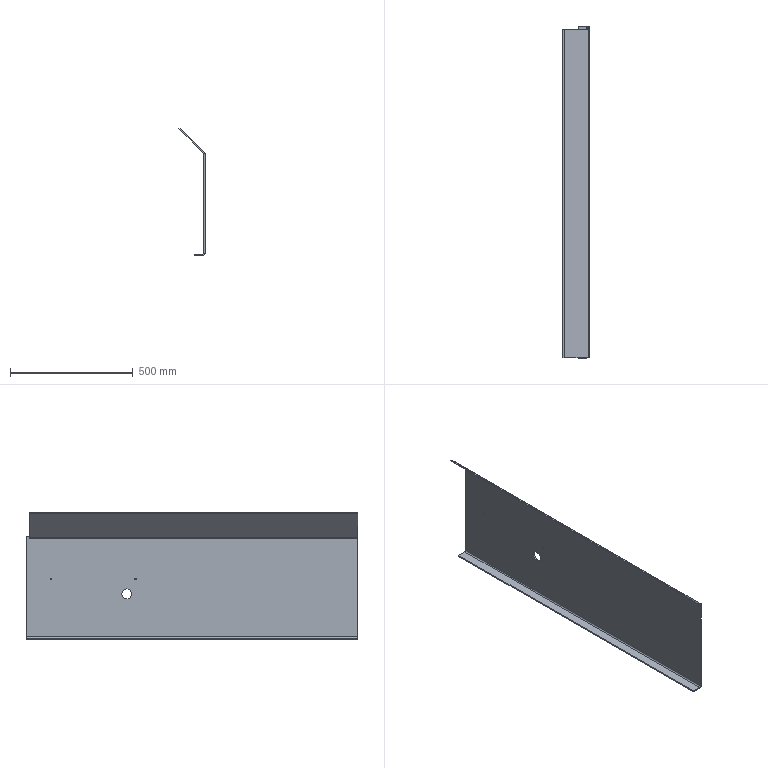Component | SolidWorks | 005FrameSheet-MetalB-1 | 2 solids | 26 faces | box 107.07 x 1350 x 515 mm | volume 3987894 mm3 | plane 16 | cylinder 10 | commonest cylinder face diameters 5 x4 40 x2 10 x2 20 x2 | material Plain Carbon Steel
build123d program:
from build123d import *

# Parameters (mm, degrees)
SKETCH2_W                  = 410
SKETCH2_H                  = 515
BOSS_EXTRUDE1_DEPTH        = 1350
FILLET1_R                  = 10
CHAMFER1_SIZE              = 100
FILLET2_R                  = 10
SHELL1_T                   = -5
CUT_EXTRUDE1_REACH         = 1461.366
SKETCH3_W                  = 320
SKETCH3_H                  = 1561.085
SKETCH7_R                  = 13
SKETCH7_R_2                = 3.25
CUT_EXTRUDE5_DEPTH         = 5
SKETCH8_R                  = 7.5
CUT_EXTRUDE6_DEPTH         = 5
M6_TAPPED_HOLE1_AT_2_COUNT = 2
M6_TAPPED_HOLE1_AT_2_PITCH = 60
LPATTERN1_COUNT            = 2
LPATTERN1_PITCH            = 345
SKETCH13_R                 = 20
CUT_EXTRUDE7_DEPTH         = 5
M6_TAPPED_HOLE3_AT_2_COUNT = 2
M6_TAPPED_HOLE3_AT_2_PITCH = 60
CUT_EXTRUDE9_DEPTH         = 1390.544
SKETCH18_W                 = 400
SKETCH18_H                 = 30
CUT_EXTRUDE10_DEPTH        = 1390.544
CUT_EXTRUDE8_DEPTH         = 1390.544
CUT_EXTRUDE8_DEPTH_BACK    = 1390.544
SKETCH16_W                 = 227.729
SKETCH16_H                 = 1450
BOSS_EXTRUDE2_DEPTH        = 1335


with BuildPart() as part:
    # Sketch2 → Boss-Extrude1 (new body)
    with BuildSketch(Plane(origin=(0, 0, 0), x_dir=(1, 0, 0), z_dir=(0, 1, 0))):
        Rectangle(SKETCH2_W, SKETCH2_H)
    extrude(amount=BOSS_EXTRUDE1_DEPTH)

    # Fillet1
    fillet1_edges = [part.edges().sort_by_distance(p)[0] for p in [
        (-205, 675, -257.5),
        (205, 675, -257.5),
    ]]
    fillet(fillet1_edges, radius=FILLET1_R)

    # Chamfer1
    chamfer1_edges = [part.edges().sort_by_distance(p)[0] for p in [
        (205, 675, 257.5),
        (-205, 675, 257.5),
    ]]
    chamfer(chamfer1_edges, length=CHAMFER1_SIZE)

    # Fillet2
    fillet2_edges = [part.edges().sort_by_distance(p)[0] for p in [
        (205, 675, 157.5),
        (-205, 675, 157.5),
    ]]
    fillet(fillet2_edges, radius=FILLET2_R)

    # Shell1
    shell1_openings = [part.faces().sort_by_distance(p)[0] for p in [
        (0, 1350, -11.096),
        (0, 0, -11.096),
        (0, 675, 257.5),
    ]]
    offset(amount=SHELL1_T, openings=shell1_openings, kind=Kind.INTERSECTION)

    # Sketch3 → Cut-Extrude1 (cut, up to next)
    with BuildSketch(Plane(origin=(0, 0, -257.5), x_dir=(-1, 0, 0), z_dir=(0, 0, -1)), mode=Mode.PRIVATE) as cut_extrude1_sk1:
        with Locations((0, 708.71)):
            Rectangle(SKETCH3_W, SKETCH3_H)
    cut_extrude1_tool1 = extrude(cut_extrude1_sk1.sketch, amount=-CUT_EXTRUDE1_REACH, mode=Mode.PRIVATE) & part.part
    add(cut_extrude1_tool1.solids().sort_by_distance((0, 708.71, -257.5))[0], mode=Mode.SUBTRACT)


with BuildPart() as cut_extrude1_piece_1:
    # of the separate pieces the step leaves, piece 1, a body of its own (cut_extrude1_pieces)
    add(part.part.solids().sort_by_distance((195, 0, -257.5))[0])

    # Sketch11 → M6 Tapped Hole2 (revolve, cut)
    with BuildSketch(Plane(origin=(205, 1250, -12.5), x_dir=(0, 0, -1), z_dir=(0, 1, 0))):
        Polygon((0, 0), (0, 16.502), (2.5, 15), (2.5, 0), align=None)
    m6_tapped_hole2 = revolve(axis=Axis((211.35, 1250, -12.5), (-1, 0, 0)), mode=Mode.SUBTRACT)

    # LPattern1: M6 Tapped Hole2 ×2
    with Locations(*[(0, -i * LPATTERN1_PITCH, 0) for i in range(1, LPATTERN1_COUNT)]):
        add(m6_tapped_hole2, mode=Mode.SUBTRACT)

    # Sketch13 → Cut-Extrude7 (cut)
    with BuildSketch(Plane(origin=(205, 0, 0), x_dir=(0, 0, -1), z_dir=(1, 0, 0))):
        with Locations((72.5, 940)):
            Circle(SKETCH13_R)
    extrude(amount=-CUT_EXTRUDE7_DEPTH, mode=Mode.SUBTRACT)


with BuildPart() as cut_extrude1_piece_2:
    # of the separate pieces the step leaves, piece 2, a body of its own (cut_extrude1_pieces)
    add(part.part.solids().sort_by_distance((-202.071, 0, 160.429))[0])

    # Sketch7 → Cut-Extrude5 (cut)
    with BuildSketch(Plane.ZY.offset(205)):
        with Locations((-151.5, 191.5)):
            Circle(SKETCH7_R)
        with Locations((-151.5, 318.5)):
            Circle(SKETCH7_R)
        with Locations((-151.5, 293)):
            Circle(SKETCH7_R_2)
        with Locations((-151.5, 217)):
            Circle(SKETCH7_R_2)
        with Locations((-93.5, 191.5)):
            Circle(SKETCH7_R)
        with Locations((-93.5, 318.5)):
            Circle(SKETCH7_R)
        with Locations((-93.5, 217)):
            Circle(SKETCH7_R_2)
        with Locations((-93.5, 293)):
            Circle(SKETCH7_R_2)
    extrude(amount=-CUT_EXTRUDE5_DEPTH, mode=Mode.SUBTRACT)

    # Sketch8 → Cut-Extrude6 (cut)
    with BuildSketch(Plane.ZY.offset(205)):
        with Locations((-147.5, 95)):
            Circle(SKETCH8_R)
        with Locations((-97.5, 95)):
            Circle(SKETCH8_R)
        with Locations((-147.5, 65)):
            Circle(SKETCH8_R)
        with Locations((-97.5, 65)):
            Circle(SKETCH8_R)
    extrude(amount=-CUT_EXTRUDE6_DEPTH, mode=Mode.SUBTRACT)

    # Sketch9 → M6 Tapped Hole1 (revolve, cut)
    with BuildSketch(Plane(origin=(-205, 80, -92.5), x_dir=(0, 0, 1), z_dir=(0, 1, 0))):
        Polygon((0, 0), (0, 16.502), (2.5, 15), (2.5, 0), align=None)
    m6_tapped_hole1 = revolve(axis=Axis((-211.35, 80, -92.5), (1, 0, 0)), mode=Mode.SUBTRACT)

    # M6 Tapped Hole1 at 2: M6 Tapped Hole1 ×2
    with Locations(*[(0, 0, -i * M6_TAPPED_HOLE1_AT_2_PITCH) for i in range(1, M6_TAPPED_HOLE1_AT_2_COUNT)]):
        add(m6_tapped_hole1, mode=Mode.SUBTRACT)

    # Sketch14 → M6 Tapped Hole3 (revolve, cut)
    with BuildSketch(Plane(origin=(-205, 1250, 100), x_dir=(0, 0, 1), z_dir=(0, 1, 0))):
        Polygon((0, 0), (0, 16.502), (2.5, 15), (2.5, 0), align=None)
    m6_tapped_hole3 = revolve(axis=Axis((-211.35, 1250, 100), (1, 0, 0)), mode=Mode.SUBTRACT)

    # M6 Tapped Hole3 at 2: M6 Tapped Hole3 ×2
    with Locations(*[(0, 0, i * M6_TAPPED_HOLE3_AT_2_PITCH) for i in range(1, M6_TAPPED_HOLE3_AT_2_COUNT)]):
        add(m6_tapped_hole3, mode=Mode.SUBTRACT)


with BuildPart() as cut_extrude9_tool:
    # Sketch17 → Cut-Extrude9 (new, through all)
    with BuildSketch(Plane(origin=(0, 1350, 0), x_dir=(1, 0, 0), z_dir=(0, 1, 0))):
        Polygon((-105, -257.5), (0, -152.5), (105, -257.5), align=None)
    extrude(amount=-CUT_EXTRUDE9_DEPTH)


with BuildPart() as cut_extrude1_piece_1_1:
    add(cut_extrude1_piece_1.part)

    # Cut-Extrude9: cut by cut_extrude9_tool
    add(cut_extrude9_tool.part, mode=Mode.SUBTRACT)


with BuildPart() as cut_extrude1_piece_2_1:
    add(cut_extrude1_piece_2.part)

    # Cut-Extrude9: cut by cut_extrude9_tool
    add(cut_extrude9_tool.part, mode=Mode.SUBTRACT)


with BuildPart() as cut_extrude10_tool:
    # Sketch18 → Cut-Extrude10 (new, through all)
    with BuildSketch(Plane.XY):
        with Locations((0, 1350)):
            Rectangle(SKETCH18_W, SKETCH18_H)
    extrude(amount=CUT_EXTRUDE10_DEPTH)


with BuildPart() as cut_extrude1_piece_1_2:
    add(cut_extrude1_piece_1_1.part)

    # Cut-Extrude10: cut by cut_extrude10_tool
    add(cut_extrude10_tool.part, mode=Mode.SUBTRACT)


with BuildPart() as cut_extrude1_piece_2_2:
    add(cut_extrude1_piece_2_1.part)

    # Cut-Extrude10: cut by cut_extrude10_tool
    add(cut_extrude10_tool.part, mode=Mode.SUBTRACT)

    # Sketch16 → Cut-Extrude8 (cut, two sides: drawn at the far end of the back side and taken through both)
    with BuildSketch(Plane.XY.offset(-CUT_EXTRUDE8_DEPTH_BACK)):
        with Locations((-113.864, 725)):
            Rectangle(SKETCH16_W, SKETCH16_H)
    extrude(amount=CUT_EXTRUDE8_DEPTH + CUT_EXTRUDE8_DEPTH_BACK, mode=Mode.SUBTRACT)


with BuildPart() as body_2:
    # Sketch19 → Boss-Extrude2 (new, through all)
    with BuildSketch(Plane(origin=(0, 1335, 0), x_dir=(1, 0, 0), z_dir=(0, 1, 0))):
        Polygon((105, -257.5), (101.464, -253.964), (97.929, -257.5), align=None)
    extrude(amount=-BOSS_EXTRUDE2_DEPTH)


solid = Compound([cut_extrude1_piece_1_2.part, body_2.part])

# Placed as in the assembly
solid = solid.moved(Location((100, 37, -262.5), (0, 0, 0)))
STEP:
#1=COLOUR_RGB('',0.7922,0.8196,0.9333);
#2=FILL_AREA_STYLE_COLOUR('',#1);
#3=FILL_AREA_STYLE('',(#2));
#4=SURFACE_STYLE_FILL_AREA(#3);
#5=SURFACE_SIDE_STYLE('',(#4));
#6=SURFACE_STYLE_USAGE(.BOTH.,#5);
#7=PRESENTATION_STYLE_ASSIGNMENT((#6));
#8=CARTESIAN_POINT('',(11.811,38.465,-12.402));
#9=VERTEX_POINT('',#8);
#10=CARTESIAN_POINT('',(11.811,38.465,-13.976));
#11=VERTEX_POINT('',#10);
#12=CARTESIAN_POINT('',(11.811,38.465,-13.189));
#13=DIRECTION('',(1.,0.,0.));
#14=DIRECTION('',(0.,0.,1.));
#15=AXIS2_PLACEMENT_3D('',#12,#13,#14);
#16=CIRCLE('',#15,0.7874);
#17=EDGE_CURVE('',#9,#11,#16,.T.);
#18=ORIENTED_EDGE('',*,*,#17,.F.);
#19=CARTESIAN_POINT('',(12.008,38.465,-12.402));
#20=VERTEX_POINT('',#19);
#21=CARTESIAN_POINT('',(-4.134,38.465,-12.402));
#22=DIRECTION('',(1.,0.,0.));
#23=VECTOR('',#22,39.37);
#24=LINE('',#21,#23);
#25=EDGE_CURVE('',#9,#20,#24,.T.);
#26=ORIENTED_EDGE('',*,*,#25,.T.);
#27=CARTESIAN_POINT('',(12.008,38.465,-13.976));
#28=VERTEX_POINT('',#27);
#29=CARTESIAN_POINT('',(12.008,38.465,-13.189));
#30=DIRECTION('',(1.,0.,0.));
#31=DIRECTION('',(0.,0.,-1.));
#32=AXIS2_PLACEMENT_3D('',#29,#30,#31);
#33=CIRCLE('',#32,0.7874);
#34=EDGE_CURVE('',#20,#28,#33,.T.);
#35=ORIENTED_EDGE('',*,*,#34,.T.);
#36=CARTESIAN_POINT('',(-4.134,38.465,-13.976));
#37=DIRECTION('',(1.,0.,0.));
#38=VECTOR('',#37,39.37);
#39=LINE('',#36,#38);
#40=EDGE_CURVE('',#11,#28,#39,.T.);
#41=ORIENTED_EDGE('',*,*,#40,.F.);
#42=EDGE_LOOP('',(#18,#26,#35,#41));
#43=FACE_OUTER_BOUND('',#42,.T.);
#44=CARTESIAN_POINT('',(-4.134,38.465,-13.189));
#45=DIRECTION('',(1.,0.,0.));
#46=DIRECTION('',(0.,0.,-1.));
#47=AXIS2_PLACEMENT_3D('',#44,#45,#46);
#48=CYLINDRICAL_SURFACE('',#47,0.7874);
#49=ADVANCED_FACE('',(#43),#48,.F.);
#50=CARTESIAN_POINT('',(11.811,37.087,-10.925));
#51=VERTEX_POINT('',#50);
#52=CARTESIAN_POINT('',(11.811,37.087,-10.728));
#53=VERTEX_POINT('',#52);
#54=CARTESIAN_POINT('',(11.811,37.087,-10.827));
#55=DIRECTION('',(-1.,0.,0.));
#56=DIRECTION('',(0.,0.,1.));
#57=AXIS2_PLACEMENT_3D('',#54,#55,#56);
#58=CIRCLE('',#57,0.09843);
#59=EDGE_CURVE('',#51,#53,#58,.T.);
#60=ORIENTED_EDGE('',*,*,#59,.T.);
#61=CARTESIAN_POINT('',(12.008,37.087,-10.728));
#62=VERTEX_POINT('',#61);
#63=CARTESIAN_POINT('',(12.008,37.087,-10.728));
#64=DIRECTION('',(1.,0.,0.));
#65=VECTOR('',#64,39.37);
#66=LINE('',#63,#65);
#67=EDGE_CURVE('',#53,#62,#66,.T.);
#68=ORIENTED_EDGE('',*,*,#67,.T.);
#69=CARTESIAN_POINT('',(12.008,37.087,-10.925));
#70=VERTEX_POINT('',#69);
#71=CARTESIAN_POINT('',(12.008,37.087,-10.827));
#72=DIRECTION('',(1.,0.,0.));
#73=DIRECTION('',(0.,0.,-1.));
#74=AXIS2_PLACEMENT_3D('',#71,#72,#73);
#75=CIRCLE('',#74,0.09843);
#76=EDGE_CURVE('',#62,#70,#75,.T.);
#77=ORIENTED_EDGE('',*,*,#76,.T.);
#78=CARTESIAN_POINT('',(12.008,37.087,-10.925));
#79=DIRECTION('',(1.,0.,0.));
#80=VECTOR('',#79,39.37);
#81=LINE('',#78,#80);
#82=EDGE_CURVE('',#51,#70,#81,.T.);
#83=ORIENTED_EDGE('',*,*,#82,.F.);
#84=EDGE_LOOP('',(#60,#68,#77,#83));
#85=FACE_OUTER_BOUND('',#84,.T.);
#86=CARTESIAN_POINT('',(12.008,37.087,-10.827));
#87=DIRECTION('',(1.,0.,0.));
#88=DIRECTION('',(0.,0.,-1.));
#89=AXIS2_PLACEMENT_3D('',#86,#87,#88);
#90=CYLINDRICAL_SURFACE('',#89,0.09843);
#91=ADVANCED_FACE('',(#85),#90,.F.);
#92=CARTESIAN_POINT('',(11.811,50.669,-10.925));
#93=VERTEX_POINT('',#92);
#94=CARTESIAN_POINT('',(11.811,50.669,-10.728));
#95=VERTEX_POINT('',#94);
#96=CARTESIAN_POINT('',(11.811,50.669,-10.827));
#97=DIRECTION('',(-1.,0.,0.));
#98=DIRECTION('',(0.,0.,1.));
#99=AXIS2_PLACEMENT_3D('',#96,#97,#98);
#100=CIRCLE('',#99,0.09843);
#101=EDGE_CURVE('',#93,#95,#100,.T.);
#102=ORIENTED_EDGE('',*,*,#101,.T.);
#103=CARTESIAN_POINT('',(12.008,50.669,-10.728));
#104=VERTEX_POINT('',#103);
#105=CARTESIAN_POINT('',(12.008,50.669,-10.728));
#106=DIRECTION('',(1.,0.,0.));
#107=VECTOR('',#106,39.37);
#108=LINE('',#105,#107);
#109=EDGE_CURVE('',#95,#104,#108,.T.);
#110=ORIENTED_EDGE('',*,*,#109,.T.);
#111=CARTESIAN_POINT('',(12.008,50.669,-10.925));
#112=VERTEX_POINT('',#111);
#113=CARTESIAN_POINT('',(12.008,50.669,-10.827));
#114=DIRECTION('',(1.,0.,0.));
#115=DIRECTION('',(0.,0.,-1.));
#116=AXIS2_PLACEMENT_3D('',#113,#114,#115);
#117=CIRCLE('',#116,0.09843);
#118=EDGE_CURVE('',#104,#112,#117,.T.);
#119=ORIENTED_EDGE('',*,*,#118,.T.);
#120=CARTESIAN_POINT('',(12.008,50.669,-10.925));
#121=DIRECTION('',(1.,0.,0.));
#122=VECTOR('',#121,39.37);
#123=LINE('',#120,#122);
#124=EDGE_CURVE('',#93,#112,#123,.T.);
#125=ORIENTED_EDGE('',*,*,#124,.F.);
#126=EDGE_LOOP('',(#102,#110,#119,#125));
#127=FACE_OUTER_BOUND('',#126,.T.);
#128=CARTESIAN_POINT('',(12.008,50.669,-10.827));
#129=DIRECTION('',(1.,0.,0.));
#130=DIRECTION('',(0.,0.,-1.));
#131=AXIS2_PLACEMENT_3D('',#128,#129,#130);
#132=CYLINDRICAL_SURFACE('',#131,0.09843);
#133=ADVANCED_FACE('',(#127),#132,.F.);
#134=CARTESIAN_POINT('',(11.811,54.606,-3.937));
#135=VERTEX_POINT('',#134);
#136=CARTESIAN_POINT('',(11.811,54.606,-20.079));
#137=VERTEX_POINT('',#136);
#138=CARTESIAN_POINT('',(11.811,54.606,-20.472));
#139=DIRECTION('',(0.,0.,-1.));
#140=VECTOR('',#139,39.37);
#141=LINE('',#138,#140);
#142=EDGE_CURVE('',#135,#137,#141,.T.);
#143=ORIENTED_EDGE('',*,*,#142,.F.);
#144=CARTESIAN_POINT('',(11.893,54.606,-4.019));
#145=VERTEX_POINT('',#144);
#146=CARTESIAN_POINT('',(12.008,54.606,-4.134));
#147=DIRECTION('',(0.7071,0.,-0.7071));
#148=VECTOR('',#147,39.37);
#149=LINE('',#146,#148);
#150=EDGE_CURVE('',#135,#145,#149,.T.);
#151=ORIENTED_EDGE('',*,*,#150,.T.);
#152=CARTESIAN_POINT('',(12.008,54.606,-4.297));
#153=VERTEX_POINT('',#152);
#154=CARTESIAN_POINT('',(11.614,54.606,-4.297));
#155=DIRECTION('',(0.,1.,0.));
#156=DIRECTION('',(-0.,0.,-1.));
#157=AXIS2_PLACEMENT_3D('',#154,#155,#156);
#158=CIRCLE('',#157,0.3937);
#159=EDGE_CURVE('',#145,#153,#158,.T.);
#160=ORIENTED_EDGE('',*,*,#159,.T.);
#161=CARTESIAN_POINT('',(12.008,54.606,-20.079));
#162=VERTEX_POINT('',#161);
#163=CARTESIAN_POINT('',(12.008,54.606,-0.1969));
#164=DIRECTION('',(0.,0.,-1.));
#165=VECTOR('',#164,39.37);
#166=LINE('',#163,#165);
#167=EDGE_CURVE('',#153,#162,#166,.T.);
#168=ORIENTED_EDGE('',*,*,#167,.T.);
#169=CARTESIAN_POINT('',(11.614,54.606,-20.472));
#170=VERTEX_POINT('',#169);
#171=CARTESIAN_POINT('',(11.614,54.606,-20.079));
#172=DIRECTION('',(0.,1.,0.));
#173=DIRECTION('',(0.,0.,-1.));
#174=AXIS2_PLACEMENT_3D('',#171,#172,#173);
#175=CIRCLE('',#174,0.3937);
#176=EDGE_CURVE('',#162,#170,#175,.T.);
#177=ORIENTED_EDGE('',*,*,#176,.T.);
#178=CARTESIAN_POINT('',(10.236,54.606,-20.472));
#179=VERTEX_POINT('',#178);
#180=CARTESIAN_POINT('',(-4.134,54.606,-20.472));
#181=DIRECTION('',(-1.,0.,0.));
#182=VECTOR('',#181,39.37);
#183=LINE('',#180,#182);
#184=EDGE_CURVE('',#170,#179,#183,.T.);
#185=ORIENTED_EDGE('',*,*,#184,.T.);
#186=CARTESIAN_POINT('',(10.236,54.606,-20.276));
#187=VERTEX_POINT('',#186);
#188=CARTESIAN_POINT('',(10.236,54.606,-0.1968));
#189=DIRECTION('',(0.,0.,-1.));
#190=VECTOR('',#189,39.37);
#191=LINE('',#188,#190);
#192=EDGE_CURVE('',#187,#179,#191,.T.);
#193=ORIENTED_EDGE('',*,*,#192,.F.);
#194=CARTESIAN_POINT('',(11.614,54.606,-20.276));
#195=VERTEX_POINT('',#194);
#196=CARTESIAN_POINT('',(12.008,54.606,-20.276));
#197=DIRECTION('',(-1.,0.,0.));
#198=VECTOR('',#197,39.37);
#199=LINE('',#196,#198);
#200=EDGE_CURVE('',#195,#187,#199,.T.);
#201=ORIENTED_EDGE('',*,*,#200,.F.);
#202=CARTESIAN_POINT('',(11.614,54.606,-20.079));
#203=DIRECTION('',(0.,1.,0.));
#204=DIRECTION('',(0.,0.,-1.));
#205=AXIS2_PLACEMENT_3D('',#202,#203,#204);
#206=CIRCLE('',#205,0.1969);
#207=EDGE_CURVE('',#137,#195,#206,.T.);
#208=ORIENTED_EDGE('',*,*,#207,.F.);
#209=EDGE_LOOP('',(#143,#151,#160,#168,#177,#185,#193,#201,#208));
#210=FACE_OUTER_BOUND('',#209,.T.);
#211=CARTESIAN_POINT('',(12.008,54.606,-20.472));
#212=DIRECTION('',(0.,-1.,0.));
#213=DIRECTION('',(0.,0.,-1.));
#214=AXIS2_PLACEMENT_3D('',#211,#212,#213);
#215=PLANE('',#214);
#216=ADVANCED_FACE('',(#210),#215,.F.);
#217=CARTESIAN_POINT('',(11.811,54.016,-3.937));
#218=VERTEX_POINT('',#217);
#219=CARTESIAN_POINT('',(11.811,54.606,-3.937));
#220=DIRECTION('',(0.,-1.,0.));
#221=VECTOR('',#220,39.37);
#222=LINE('',#219,#221);
#223=EDGE_CURVE('',#135,#218,#222,.T.);
#224=ORIENTED_EDGE('',*,*,#223,.T.);
#225=CARTESIAN_POINT('',(8.071,54.016,-0.1969));
#226=VERTEX_POINT('',#225);
#227=CARTESIAN_POINT('',(12.008,54.016,-4.134));
#228=DIRECTION('',(-0.7071,0.,0.7071));
#229=VECTOR('',#228,39.37);
#230=LINE('',#227,#229);
#231=EDGE_CURVE('',#218,#226,#230,.T.);
#232=ORIENTED_EDGE('',*,*,#231,.T.);
#233=CARTESIAN_POINT('',(8.071,1.457,-0.1969));
#234=VERTEX_POINT('',#233);
#235=CARTESIAN_POINT('',(8.071,54.606,-0.1969));
#236=DIRECTION('',(0.,1.,0.));
#237=VECTOR('',#236,39.37);
#238=LINE('',#235,#237);
#239=EDGE_CURVE('',#234,#226,#238,.T.);
#240=ORIENTED_EDGE('',*,*,#239,.F.);
#241=CARTESIAN_POINT('',(11.893,1.457,-4.019));
#242=VERTEX_POINT('',#241);
#243=CARTESIAN_POINT('',(20.177,1.457,-12.303));
#244=DIRECTION('',(-0.7071,0.,0.7071));
#245=VECTOR('',#244,39.37);
#246=LINE('',#243,#245);
#247=EDGE_CURVE('',#242,#234,#246,.T.);
#248=ORIENTED_EDGE('',*,*,#247,.F.);
#249=CARTESIAN_POINT('',(11.893,54.606,-4.019));
#250=DIRECTION('',(0.,1.,0.));
#251=VECTOR('',#250,39.37);
#252=LINE('',#249,#251);
#253=EDGE_CURVE('',#242,#145,#252,.T.);
#254=ORIENTED_EDGE('',*,*,#253,.T.);
#255=ORIENTED_EDGE('',*,*,#150,.F.);
#256=EDGE_LOOP('',(#224,#232,#240,#248,#254,#255));
#257=FACE_OUTER_BOUND('',#256,.T.);
#258=CARTESIAN_POINT('',(12.008,54.606,-4.134));
#259=DIRECTION('',(-0.7071,0.,-0.7071));
#260=DIRECTION('',(-0.7071,0.,0.7071));
#261=AXIS2_PLACEMENT_3D('',#258,#259,#260);
#262=PLANE('',#261);
#263=ADVANCED_FACE('',(#257),#262,.F.);
#264=CARTESIAN_POINT('',(11.753,54.016,-4.158));
#265=VERTEX_POINT('',#264);
#266=CARTESIAN_POINT('',(7.932,54.016,-0.336));
#267=VERTEX_POINT('',#266);
#268=CARTESIAN_POINT('',(11.869,54.016,-4.273));
#269=DIRECTION('',(-0.7071,0.,0.7071));
#270=VECTOR('',#269,39.37);
#271=LINE('',#268,#270);
#272=EDGE_CURVE('',#265,#267,#271,.T.);
#273=ORIENTED_EDGE('',*,*,#272,.F.);
#274=CARTESIAN_POINT('',(11.753,1.457,-4.158));
#275=VERTEX_POINT('',#274);
#276=CARTESIAN_POINT('',(11.753,54.606,-4.158));
#277=DIRECTION('',(0.,1.,0.));
#278=VECTOR('',#277,39.37);
#279=LINE('',#276,#278);
#280=EDGE_CURVE('',#275,#265,#279,.T.);
#281=ORIENTED_EDGE('',*,*,#280,.F.);
#282=CARTESIAN_POINT('',(7.932,1.457,-0.336));
#283=VERTEX_POINT('',#282);
#284=CARTESIAN_POINT('',(20.038,1.457,-12.442));
#285=DIRECTION('',(-0.7071,0.,0.7071));
#286=VECTOR('',#285,39.37);
#287=LINE('',#284,#286);
#288=EDGE_CURVE('',#275,#283,#287,.T.);
#289=ORIENTED_EDGE('',*,*,#288,.T.);
#290=CARTESIAN_POINT('',(7.932,54.606,-0.336));
#291=DIRECTION('',(0.,1.,0.));
#292=VECTOR('',#291,39.37);
#293=LINE('',#290,#292);
#294=EDGE_CURVE('',#283,#267,#293,.T.);
#295=ORIENTED_EDGE('',*,*,#294,.T.);
#296=EDGE_LOOP('',(#273,#281,#289,#295));
#297=FACE_OUTER_BOUND('',#296,.T.);
#298=CARTESIAN_POINT('',(11.869,54.606,-4.273));
#299=DIRECTION('',(-0.7071,0.,-0.7071));
#300=DIRECTION('',(-0.7071,0.,0.7071));
#301=AXIS2_PLACEMENT_3D('',#298,#299,#300);
#302=PLANE('',#301);
#303=ADVANCED_FACE('',(#297),#302,.T.);
#304=CARTESIAN_POINT('',(11.811,54.016,-4.297));
#305=VERTEX_POINT('',#304);
#306=CARTESIAN_POINT('',(11.614,54.016,-4.297));
#307=DIRECTION('',(0.,-1.,0.));
#308=DIRECTION('',(0.,0.,1.));
#309=AXIS2_PLACEMENT_3D('',#306,#307,#308);
#310=CIRCLE('',#309,0.1969);
#311=EDGE_CURVE('',#305,#265,#310,.T.);
#312=ORIENTED_EDGE('',*,*,#311,.F.);
#313=CARTESIAN_POINT('',(11.811,1.457,-4.297));
#314=VERTEX_POINT('',#313);
#315=CARTESIAN_POINT('',(11.811,54.606,-4.297));
#316=DIRECTION('',(0.,-1.,0.));
#317=VECTOR('',#316,39.37);
#318=LINE('',#315,#317);
#319=EDGE_CURVE('',#305,#314,#318,.T.);
#320=ORIENTED_EDGE('',*,*,#319,.T.);
#321=CARTESIAN_POINT('',(11.614,1.457,-4.297));
#322=DIRECTION('',(0.,-1.,0.));
#323=DIRECTION('',(0.,0.,-1.));
#324=AXIS2_PLACEMENT_3D('',#321,#322,#323);
#325=CIRCLE('',#324,0.1969);
#326=EDGE_CURVE('',#314,#275,#325,.T.);
#327=ORIENTED_EDGE('',*,*,#326,.T.);
#328=ORIENTED_EDGE('',*,*,#280,.T.);
#329=EDGE_LOOP('',(#312,#320,#327,#328));
#330=FACE_OUTER_BOUND('',#329,.T.);
#331=CARTESIAN_POINT('',(11.614,54.606,-4.297));
#332=DIRECTION('',(0.,-1.,0.));
#333=DIRECTION('',(0.,0.,-1.));
#334=AXIS2_PLACEMENT_3D('',#331,#332,#333);
#335=CYLINDRICAL_SURFACE('',#334,0.1969);
#336=ADVANCED_FACE('',(#330),#335,.F.);
#337=CARTESIAN_POINT('',(3.937,54.016,-4.331));
#338=DIRECTION('',(0.7071,0.,0.7071));
#339=VECTOR('',#338,39.37);
#340=LINE('',#337,#339);
#341=EDGE_CURVE('',#267,#226,#340,.T.);
#342=ORIENTED_EDGE('',*,*,#341,.F.);
#343=ORIENTED_EDGE('',*,*,#294,.F.);
#344=CARTESIAN_POINT('',(3.937,1.457,-4.331));
#345=DIRECTION('',(-0.7071,0.,-0.7071));
#346=VECTOR('',#345,39.37);
#347=LINE('',#344,#346);
#348=EDGE_CURVE('',#234,#283,#347,.T.);
#349=ORIENTED_EDGE('',*,*,#348,.F.);
#350=ORIENTED_EDGE('',*,*,#239,.T.);
#351=EDGE_LOOP('',(#342,#343,#349,#350));
#352=FACE_OUTER_BOUND('',#351,.T.);
#353=CARTESIAN_POINT('',(3.937,1.457,-4.331));
#354=DIRECTION('',(0.7071,0.,-0.7071));
#355=DIRECTION('',(-0.7071,0.,-0.7071));
#356=AXIS2_PLACEMENT_3D('',#353,#354,#355);
#357=PLANE('',#356);
#358=ADVANCED_FACE('',(#352),#357,.F.);
#359=CARTESIAN_POINT('',(11.614,1.457,-20.472));
#360=VERTEX_POINT('',#359);
#361=CARTESIAN_POINT('',(10.236,1.457,-20.472));
#362=VERTEX_POINT('',#361);
#363=CARTESIAN_POINT('',(-4.134,1.457,-20.472));
#364=DIRECTION('',(-1.,0.,0.));
#365=VECTOR('',#364,39.37);
#366=LINE('',#363,#365);
#367=EDGE_CURVE('',#360,#362,#366,.T.);
#368=ORIENTED_EDGE('',*,*,#367,.T.);
#369=CARTESIAN_POINT('',(10.236,60.089,-20.472));
#370=DIRECTION('',(-0.,-1.,0.));
#371=VECTOR('',#370,39.37);
#372=LINE('',#369,#371);
#373=EDGE_CURVE('',#179,#362,#372,.T.);
#374=ORIENTED_EDGE('',*,*,#373,.F.);
#375=ORIENTED_EDGE('',*,*,#184,.F.);
#376=CARTESIAN_POINT('',(11.614,54.606,-20.472));
#377=DIRECTION('',(0.,-1.,0.));
#378=VECTOR('',#377,39.37);
#379=LINE('',#376,#378);
#380=EDGE_CURVE('',#170,#360,#379,.T.);
#381=ORIENTED_EDGE('',*,*,#380,.T.);
#382=EDGE_LOOP('',(#368,#374,#375,#381));
#383=FACE_OUTER_BOUND('',#382,.T.);
#384=CARTESIAN_POINT('',(-4.134,54.606,-20.472));
#385=DIRECTION('',(0.,0.,1.));
#386=DIRECTION('',(1.,0.,0.));
#387=AXIS2_PLACEMENT_3D('',#384,#385,#386);
#388=PLANE('',#387);
#389=ADVANCED_FACE('',(#383),#388,.F.);
#390=ORIENTED_EDGE('',*,*,#348,.T.);
#391=ORIENTED_EDGE('',*,*,#288,.F.);
#392=ORIENTED_EDGE('',*,*,#326,.F.);
#393=CARTESIAN_POINT('',(11.811,1.457,-20.079));
#394=VERTEX_POINT('',#393);
#395=CARTESIAN_POINT('',(11.811,1.457,-20.472));
#396=DIRECTION('',(0.,0.,-1.));
#397=VECTOR('',#396,39.37);
#398=LINE('',#395,#397);
#399=EDGE_CURVE('',#314,#394,#398,.T.);
#400=ORIENTED_EDGE('',*,*,#399,.T.);
#401=CARTESIAN_POINT('',(11.614,1.457,-20.276));
#402=VERTEX_POINT('',#401);
#403=CARTESIAN_POINT('',(11.614,1.457,-20.079));
#404=DIRECTION('',(0.,-1.,0.));
#405=DIRECTION('',(0.,0.,-1.));
#406=AXIS2_PLACEMENT_3D('',#403,#404,#405);
#407=CIRCLE('',#406,0.1969);
#408=EDGE_CURVE('',#402,#394,#407,.T.);
#409=ORIENTED_EDGE('',*,*,#408,.F.);
#410=CARTESIAN_POINT('',(10.236,1.457,-20.276));
#411=VERTEX_POINT('',#410);
#412=CARTESIAN_POINT('',(12.008,1.457,-20.276));
#413=DIRECTION('',(-1.,0.,0.));
#414=VECTOR('',#413,39.37);
#415=LINE('',#412,#414);
#416=EDGE_CURVE('',#402,#411,#415,.T.);
#417=ORIENTED_EDGE('',*,*,#416,.T.);
#418=CARTESIAN_POINT('',(10.236,1.457,-0.1968));
#419=DIRECTION('',(0.,0.,-1.));
#420=VECTOR('',#419,39.37);
#421=LINE('',#418,#420);
#422=EDGE_CURVE('',#411,#362,#421,.T.);
#423=ORIENTED_EDGE('',*,*,#422,.T.);
#424=ORIENTED_EDGE('',*,*,#367,.F.);
#425=CARTESIAN_POINT('',(12.008,1.457,-20.079));
#426=VERTEX_POINT('',#425);
#427=CARTESIAN_POINT('',(11.614,1.457,-20.079));
#428=DIRECTION('',(0.,-1.,0.));
#429=DIRECTION('',(0.,0.,-1.));
#430=AXIS2_PLACEMENT_3D('',#427,#428,#429);
#431=CIRCLE('',#430,0.3937);
#432=EDGE_CURVE('',#360,#426,#431,.T.);
#433=ORIENTED_EDGE('',*,*,#432,.T.);
#434=CARTESIAN_POINT('',(12.008,1.457,-4.297));
#435=VERTEX_POINT('',#434);
#436=CARTESIAN_POINT('',(12.008,1.457,-0.1969));
#437=DIRECTION('',(0.,0.,-1.));
#438=VECTOR('',#437,39.37);
#439=LINE('',#436,#438);
#440=EDGE_CURVE('',#435,#426,#439,.T.);
#441=ORIENTED_EDGE('',*,*,#440,.F.);
#442=CARTESIAN_POINT('',(11.614,1.457,-4.297));
#443=DIRECTION('',(0.,-1.,0.));
#444=DIRECTION('',(0.,0.,-1.));
#445=AXIS2_PLACEMENT_3D('',#442,#443,#444);
#446=CIRCLE('',#445,0.3937);
#447=EDGE_CURVE('',#435,#242,#446,.T.);
#448=ORIENTED_EDGE('',*,*,#447,.T.);
#449=ORIENTED_EDGE('',*,*,#247,.T.);
#450=EDGE_LOOP('',(#390,#391,#392,#400,#409,#417,#423,#424,#433,#441,#448,#449));
#451=FACE_OUTER_BOUND('',#450,.T.);
#452=CARTESIAN_POINT('',(12.008,1.457,-20.472));
#453=DIRECTION('',(0.,-1.,0.));
#454=DIRECTION('',(0.,0.,-1.));
#455=AXIS2_PLACEMENT_3D('',#452,#453,#454);
#456=PLANE('',#455);
#457=ADVANCED_FACE('',(#451),#456,.T.);
#458=CARTESIAN_POINT('',(10.236,60.089,-20.276));
#459=DIRECTION('',(-0.,-1.,0.));
#460=VECTOR('',#459,39.37);
#461=LINE('',#458,#460);
#462=EDGE_CURVE('',#187,#411,#461,.T.);
#463=ORIENTED_EDGE('',*,*,#462,.T.);
#464=ORIENTED_EDGE('',*,*,#416,.F.);
#465=CARTESIAN_POINT('',(11.614,54.606,-20.276));
#466=DIRECTION('',(0.,-1.,0.));
#467=VECTOR('',#466,39.37);
#468=LINE('',#465,#467);
#469=EDGE_CURVE('',#195,#402,#468,.T.);
#470=ORIENTED_EDGE('',*,*,#469,.F.);
#471=ORIENTED_EDGE('',*,*,#200,.T.);
#472=EDGE_LOOP('',(#463,#464,#470,#471));
#473=FACE_OUTER_BOUND('',#472,.T.);
#474=CARTESIAN_POINT('',(-4.134,54.606,-20.276));
#475=DIRECTION('',(0.,0.,1.));
#476=DIRECTION('',(1.,0.,0.));
#477=AXIS2_PLACEMENT_3D('',#474,#475,#476);
#478=PLANE('',#477);
#479=ADVANCED_FACE('',(#473),#478,.T.);
#480=CARTESIAN_POINT('',(12.008,38.465,-13.189));
#481=DIRECTION('',(1.,0.,0.));
#482=DIRECTION('',(0.,0.,-1.));
#483=AXIS2_PLACEMENT_3D('',#480,#481,#482);
#484=CIRCLE('',#483,0.7874);
#485=EDGE_CURVE('',#28,#20,#484,.T.);
#486=ORIENTED_EDGE('',*,*,#485,.F.);
#487=ORIENTED_EDGE('',*,*,#34,.F.);
#488=EDGE_LOOP('',(#486,#487));
#489=FACE_BOUND('',#488,.T.);
#490=CARTESIAN_POINT('',(12.008,37.087,-10.827));
#491=DIRECTION('',(1.,0.,0.));
#492=DIRECTION('',(0.,0.,-1.));
#493=AXIS2_PLACEMENT_3D('',#490,#491,#492);
#494=CIRCLE('',#493,0.09843);
#495=EDGE_CURVE('',#70,#62,#494,.T.);
#496=ORIENTED_EDGE('',*,*,#495,.F.);
#497=ORIENTED_EDGE('',*,*,#76,.F.);
#498=EDGE_LOOP('',(#496,#497));
#499=FACE_BOUND('',#498,.T.);
#500=CARTESIAN_POINT('',(12.008,50.669,-10.827));
#501=DIRECTION('',(1.,0.,0.));
#502=DIRECTION('',(0.,0.,-1.));
#503=AXIS2_PLACEMENT_3D('',#500,#501,#502);
#504=CIRCLE('',#503,0.09843);
#505=EDGE_CURVE('',#112,#104,#504,.T.);
#506=ORIENTED_EDGE('',*,*,#505,.F.);
#507=ORIENTED_EDGE('',*,*,#118,.F.);
#508=EDGE_LOOP('',(#506,#507));
#509=FACE_BOUND('',#508,.T.);
#510=ORIENTED_EDGE('',*,*,#167,.F.);
#511=CARTESIAN_POINT('',(12.008,1.457,-4.297));
#512=DIRECTION('',(0.,-1.,0.));
#513=VECTOR('',#512,39.37);
#514=LINE('',#511,#513);
#515=EDGE_CURVE('',#153,#435,#514,.T.);
#516=ORIENTED_EDGE('',*,*,#515,.T.);
#517=ORIENTED_EDGE('',*,*,#440,.T.);
#518=CARTESIAN_POINT('',(12.008,54.606,-20.079));
#519=DIRECTION('',(0.,1.,0.));
#520=VECTOR('',#519,39.37);
#521=LINE('',#518,#520);
#522=EDGE_CURVE('',#426,#162,#521,.T.);
#523=ORIENTED_EDGE('',*,*,#522,.T.);
#524=EDGE_LOOP('',(#510,#516,#517,#523));
#525=FACE_OUTER_BOUND('',#524,.T.);
#526=CARTESIAN_POINT('',(12.008,54.606,-0.1969));
#527=DIRECTION('',(-1.,0.,0.));
#528=DIRECTION('',(0.,0.,1.));
#529=AXIS2_PLACEMENT_3D('',#526,#527,#528);
#530=PLANE('',#529);
#531=ADVANCED_FACE('',(#489,#499,#509,#525),#530,.F.);
#532=ORIENTED_EDGE('',*,*,#176,.F.);
#533=ORIENTED_EDGE('',*,*,#522,.F.);
#534=ORIENTED_EDGE('',*,*,#432,.F.);
#535=ORIENTED_EDGE('',*,*,#380,.F.);
#536=EDGE_LOOP('',(#532,#533,#534,#535));
#537=FACE_OUTER_BOUND('',#536,.T.);
#538=CARTESIAN_POINT('',(11.614,54.606,-20.079));
#539=DIRECTION('',(0.,-1.,0.));
#540=DIRECTION('',(0.,0.,-1.));
#541=AXIS2_PLACEMENT_3D('',#538,#539,#540);
#542=CYLINDRICAL_SURFACE('',#541,0.3937);
#543=ADVANCED_FACE('',(#537),#542,.T.);
#544=ORIENTED_EDGE('',*,*,#159,.F.);
#545=ORIENTED_EDGE('',*,*,#253,.F.);
#546=ORIENTED_EDGE('',*,*,#447,.F.);
#547=ORIENTED_EDGE('',*,*,#515,.F.);
#548=EDGE_LOOP('',(#544,#545,#546,#547));
#549=FACE_OUTER_BOUND('',#548,.T.);
#550=CARTESIAN_POINT('',(11.614,54.606,-4.297));
#551=DIRECTION('',(0.,-1.,0.));
#552=DIRECTION('',(0.,0.,-1.));
#553=AXIS2_PLACEMENT_3D('',#550,#551,#552);
#554=CYLINDRICAL_SURFACE('',#553,0.3937);
#555=ADVANCED_FACE('',(#549),#554,.T.);
#556=ORIENTED_EDGE('',*,*,#319,.F.);
#557=CARTESIAN_POINT('',(11.811,54.016,-0.1969));
#558=DIRECTION('',(0.,0.,-1.));
#559=VECTOR('',#558,39.37);
#560=LINE('',#557,#559);
#561=EDGE_CURVE('',#218,#305,#560,.T.);
#562=ORIENTED_EDGE('',*,*,#561,.F.);
#563=ORIENTED_EDGE('',*,*,#223,.F.);
#564=ORIENTED_EDGE('',*,*,#142,.T.);
#565=CARTESIAN_POINT('',(11.811,54.606,-20.079));
#566=DIRECTION('',(0.,1.,0.));
#567=VECTOR('',#566,39.37);
#568=LINE('',#565,#567);
#569=EDGE_CURVE('',#394,#137,#568,.T.);
#570=ORIENTED_EDGE('',*,*,#569,.F.);
#571=ORIENTED_EDGE('',*,*,#399,.F.);
#572=EDGE_LOOP('',(#556,#562,#563,#564,#570,#571));
#573=FACE_OUTER_BOUND('',#572,.T.);
#574=CARTESIAN_POINT('',(11.811,38.465,-13.189));
#575=DIRECTION('',(1.,0.,0.));
#576=DIRECTION('',(0.,0.,1.));
#577=AXIS2_PLACEMENT_3D('',#574,#575,#576);
#578=CIRCLE('',#577,0.7874);
#579=EDGE_CURVE('',#11,#9,#578,.T.);
#580=ORIENTED_EDGE('',*,*,#579,.T.);
#581=ORIENTED_EDGE('',*,*,#17,.T.);
#582=EDGE_LOOP('',(#580,#581));
#583=FACE_BOUND('',#582,.T.);
#584=ORIENTED_EDGE('',*,*,#59,.F.);
#585=CARTESIAN_POINT('',(11.811,37.087,-10.827));
#586=DIRECTION('',(-1.,0.,0.));
#587=DIRECTION('',(0.,0.,1.));
#588=AXIS2_PLACEMENT_3D('',#585,#586,#587);
#589=CIRCLE('',#588,0.09843);
#590=EDGE_CURVE('',#53,#51,#589,.T.);
#591=ORIENTED_EDGE('',*,*,#590,.F.);
#592=EDGE_LOOP('',(#584,#591));
#593=FACE_BOUND('',#592,.T.);
#594=ORIENTED_EDGE('',*,*,#101,.F.);
#595=CARTESIAN_POINT('',(11.811,50.669,-10.827));
#596=DIRECTION('',(-1.,0.,0.));
#597=DIRECTION('',(0.,0.,1.));
#598=AXIS2_PLACEMENT_3D('',#595,#596,#597);
#599=CIRCLE('',#598,0.09843);
#600=EDGE_CURVE('',#95,#93,#599,.T.);
#601=ORIENTED_EDGE('',*,*,#600,.F.);
#602=EDGE_LOOP('',(#594,#601));
#603=FACE_BOUND('',#602,.T.);
#604=CARTESIAN_POINT('',(11.811,54.606,-0.1969));
#605=DIRECTION('',(-1.,0.,0.));
#606=DIRECTION('',(0.,0.,1.));
#607=AXIS2_PLACEMENT_3D('',#604,#605,#606);
#608=PLANE('',#607);
#609=ADVANCED_FACE('',(#573,#583,#593,#603),#608,.T.);
#610=ORIENTED_EDGE('',*,*,#207,.T.);
#611=ORIENTED_EDGE('',*,*,#469,.T.);
#612=ORIENTED_EDGE('',*,*,#408,.T.);
#613=ORIENTED_EDGE('',*,*,#569,.T.);
#614=EDGE_LOOP('',(#610,#611,#612,#613));
#615=FACE_OUTER_BOUND('',#614,.T.);
#616=CARTESIAN_POINT('',(11.614,54.606,-20.079));
#617=DIRECTION('',(0.,-1.,0.));
#618=DIRECTION('',(0.,0.,-1.));
#619=AXIS2_PLACEMENT_3D('',#616,#617,#618);
#620=CYLINDRICAL_SURFACE('',#619,0.1969);
#621=ADVANCED_FACE('',(#615),#620,.F.);
#622=ORIENTED_EDGE('',*,*,#192,.T.);
#623=ORIENTED_EDGE('',*,*,#373,.T.);
#624=ORIENTED_EDGE('',*,*,#422,.F.);
#625=ORIENTED_EDGE('',*,*,#462,.F.);
#626=EDGE_LOOP('',(#622,#623,#624,#625));
#627=FACE_OUTER_BOUND('',#626,.T.);
#628=CARTESIAN_POINT('',(10.236,60.089,-0.1968));
#629=DIRECTION('',(1.,-0.,0.));
#630=DIRECTION('',(0.,1.,0.));
#631=AXIS2_PLACEMENT_3D('',#628,#629,#630);
#632=PLANE('',#631);
#633=ADVANCED_FACE('',(#627),#632,.F.);
#634=ORIENTED_EDGE('',*,*,#109,.F.);
#635=ORIENTED_EDGE('',*,*,#600,.T.);
#636=ORIENTED_EDGE('',*,*,#124,.T.);
#637=ORIENTED_EDGE('',*,*,#505,.T.);
#638=EDGE_LOOP('',(#634,#635,#636,#637));
#639=FACE_OUTER_BOUND('',#638,.T.);
#640=CARTESIAN_POINT('',(12.008,50.669,-10.827));
#641=DIRECTION('',(1.,0.,0.));
#642=DIRECTION('',(0.,0.,-1.));
#643=AXIS2_PLACEMENT_3D('',#640,#641,#642);
#644=CYLINDRICAL_SURFACE('',#643,0.09843);
#645=ADVANCED_FACE('',(#639),#644,.F.);
#646=ORIENTED_EDGE('',*,*,#67,.F.);
#647=ORIENTED_EDGE('',*,*,#590,.T.);
#648=ORIENTED_EDGE('',*,*,#82,.T.);
#649=ORIENTED_EDGE('',*,*,#495,.T.);
#650=EDGE_LOOP('',(#646,#647,#648,#649));
#651=FACE_OUTER_BOUND('',#650,.T.);
#652=CARTESIAN_POINT('',(12.008,37.087,-10.827));
#653=DIRECTION('',(1.,0.,0.));
#654=DIRECTION('',(0.,0.,-1.));
#655=AXIS2_PLACEMENT_3D('',#652,#653,#654);
#656=CYLINDRICAL_SURFACE('',#655,0.09843);
#657=ADVANCED_FACE('',(#651),#656,.F.);
#658=ORIENTED_EDGE('',*,*,#25,.F.);
#659=ORIENTED_EDGE('',*,*,#579,.F.);
#660=ORIENTED_EDGE('',*,*,#40,.T.);
#661=ORIENTED_EDGE('',*,*,#485,.T.);
#662=EDGE_LOOP('',(#658,#659,#660,#661));
#663=FACE_OUTER_BOUND('',#662,.T.);
#664=CARTESIAN_POINT('',(-4.134,38.465,-13.189));
#665=DIRECTION('',(1.,0.,0.));
#666=DIRECTION('',(0.,0.,-1.));
#667=AXIS2_PLACEMENT_3D('',#664,#665,#666);
#668=CYLINDRICAL_SURFACE('',#667,0.7874);
#669=ADVANCED_FACE('',(#663),#668,.F.);
#670=ORIENTED_EDGE('',*,*,#311,.T.);
#671=ORIENTED_EDGE('',*,*,#272,.T.);
#672=ORIENTED_EDGE('',*,*,#341,.T.);
#673=ORIENTED_EDGE('',*,*,#231,.F.);
#674=ORIENTED_EDGE('',*,*,#561,.T.);
#675=EDGE_LOOP('',(#670,#671,#672,#673,#674));
#676=FACE_OUTER_BOUND('',#675,.T.);
#677=CARTESIAN_POINT('',(-3.937,54.016,-0.1969));
#678=DIRECTION('',(0.,1.,0.));
#679=DIRECTION('',(0.,0.,1.));
#680=AXIS2_PLACEMENT_3D('',#677,#678,#679);
#681=PLANE('',#680);
#682=ADVANCED_FACE('',(#676),#681,.T.);
#683=CLOSED_SHELL('',(#49,#91,#133,#216,#263,#303,#336,#358,#389,#457,#479,#531,#543,#555,#609,#621,#633,#645,#657,#669,#682));
#684=MANIFOLD_SOLID_BREP('',#683);
#685=STYLED_ITEM('',(#7),#684);
#686=PRESENTATION_LAYER_ASSIGNMENT('','',(#685));
#687=COLOUR_RGB('',0.7922,0.8196,0.9333);
#688=FILL_AREA_STYLE_COLOUR('',#687);
#689=FILL_AREA_STYLE('',(#688));
#690=SURFACE_STYLE_FILL_AREA(#689);
#691=SURFACE_SIDE_STYLE('',(#690));
#692=SURFACE_STYLE_USAGE(.BOTH.,#691);
#693=PRESENTATION_STYLE_ASSIGNMENT((#692));
#694=CARTESIAN_POINT('',(7.792,54.016,-0.1969));
#695=VERTEX_POINT('',#694);
#696=CARTESIAN_POINT('',(8.071,54.016,-0.1969));
#697=VERTEX_POINT('',#696);
#698=CARTESIAN_POINT('',(7.792,54.016,-0.1969));
#699=DIRECTION('',(1.,0.,0.));
#700=VECTOR('',#699,39.37);
#701=LINE('',#698,#700);
#702=EDGE_CURVE('',#695,#697,#701,.T.);
#703=ORIENTED_EDGE('',*,*,#702,.F.);
#704=CARTESIAN_POINT('',(7.792,1.457,-0.1969));
#705=VERTEX_POINT('',#704);
#706=CARTESIAN_POINT('',(7.792,1.457,-0.1969));
#707=DIRECTION('',(0.,1.,0.));
#708=VECTOR('',#707,39.37);
#709=LINE('',#706,#708);
#710=EDGE_CURVE('',#705,#695,#709,.T.);
#711=ORIENTED_EDGE('',*,*,#710,.F.);
#712=CARTESIAN_POINT('',(8.071,1.457,-0.1969));
#713=VERTEX_POINT('',#712);
#714=CARTESIAN_POINT('',(7.792,1.457,-0.1969));
#715=DIRECTION('',(1.,0.,0.));
#716=VECTOR('',#715,39.37);
#717=LINE('',#714,#716);
#718=EDGE_CURVE('',#705,#713,#717,.T.);
#719=ORIENTED_EDGE('',*,*,#718,.T.);
#720=CARTESIAN_POINT('',(8.071,1.457,-0.1969));
#721=DIRECTION('',(0.,1.,0.));
#722=VECTOR('',#721,39.37);
#723=LINE('',#720,#722);
#724=EDGE_CURVE('',#713,#697,#723,.T.);
#725=ORIENTED_EDGE('',*,*,#724,.T.);
#726=EDGE_LOOP('',(#703,#711,#719,#725));
#727=FACE_OUTER_BOUND('',#726,.T.);
#728=CARTESIAN_POINT('',(7.792,1.457,-0.1969));
#729=DIRECTION('',(0.,0.,1.));
#730=DIRECTION('',(1.,0.,0.));
#731=AXIS2_PLACEMENT_3D('',#728,#729,#730);
#732=PLANE('',#731);
#733=ADVANCED_FACE('',(#727),#732,.T.);
#734=CARTESIAN_POINT('',(7.932,54.016,-0.336));
#735=VERTEX_POINT('',#734);
#736=CARTESIAN_POINT('',(7.932,54.016,-0.336));
#737=DIRECTION('',(-0.7071,0.,0.7071));
#738=VECTOR('',#737,39.37);
#739=LINE('',#736,#738);
#740=EDGE_CURVE('',#735,#695,#739,.T.);
#741=ORIENTED_EDGE('',*,*,#740,.F.);
#742=CARTESIAN_POINT('',(7.932,1.457,-0.336));
#743=VERTEX_POINT('',#742);
#744=CARTESIAN_POINT('',(7.932,1.457,-0.336));
#745=DIRECTION('',(0.,1.,0.));
#746=VECTOR('',#745,39.37);
#747=LINE('',#744,#746);
#748=EDGE_CURVE('',#743,#735,#747,.T.);
#749=ORIENTED_EDGE('',*,*,#748,.F.);
#750=CARTESIAN_POINT('',(7.932,1.457,-0.336));
#751=DIRECTION('',(-0.7071,0.,0.7071));
#752=VECTOR('',#751,39.37);
#753=LINE('',#750,#752);
#754=EDGE_CURVE('',#743,#705,#753,.T.);
#755=ORIENTED_EDGE('',*,*,#754,.T.);
#756=ORIENTED_EDGE('',*,*,#710,.T.);
#757=EDGE_LOOP('',(#741,#749,#755,#756));
#758=FACE_OUTER_BOUND('',#757,.T.);
#759=CARTESIAN_POINT('',(7.932,1.457,-0.336));
#760=DIRECTION('',(-0.7071,0.,-0.7071));
#761=DIRECTION('',(-0.7071,0.,0.7071));
#762=AXIS2_PLACEMENT_3D('',#759,#760,#761);
#763=PLANE('',#762);
#764=ADVANCED_FACE('',(#758),#763,.T.);
#765=CARTESIAN_POINT('',(8.071,54.016,-0.1969));
#766=DIRECTION('',(-0.7071,0.,-0.7071));
#767=VECTOR('',#766,39.37);
#768=LINE('',#765,#767);
#769=EDGE_CURVE('',#697,#735,#768,.T.);
#770=ORIENTED_EDGE('',*,*,#769,.F.);
#771=ORIENTED_EDGE('',*,*,#724,.F.);
#772=CARTESIAN_POINT('',(8.071,1.457,-0.1969));
#773=DIRECTION('',(-0.7071,0.,-0.7071));
#774=VECTOR('',#773,39.37);
#775=LINE('',#772,#774);
#776=EDGE_CURVE('',#713,#743,#775,.T.);
#777=ORIENTED_EDGE('',*,*,#776,.T.);
#778=ORIENTED_EDGE('',*,*,#748,.T.);
#779=EDGE_LOOP('',(#770,#771,#777,#778));
#780=FACE_OUTER_BOUND('',#779,.T.);
#781=CARTESIAN_POINT('',(8.071,1.457,-0.1969));
#782=DIRECTION('',(0.7071,0.,-0.7071));
#783=DIRECTION('',(-0.7071,0.,-0.7071));
#784=AXIS2_PLACEMENT_3D('',#781,#782,#783);
#785=PLANE('',#784);
#786=ADVANCED_FACE('',(#780),#785,.T.);
#787=ORIENTED_EDGE('',*,*,#718,.F.);
#788=ORIENTED_EDGE('',*,*,#754,.F.);
#789=ORIENTED_EDGE('',*,*,#776,.F.);
#790=EDGE_LOOP('',(#787,#788,#789));
#791=FACE_OUTER_BOUND('',#790,.T.);
#792=CARTESIAN_POINT('',(8.071,1.457,-0.1969));
#793=DIRECTION('',(0.,1.,0.));
#794=DIRECTION('',(0.,0.,1.));
#795=AXIS2_PLACEMENT_3D('',#792,#793,#794);
#796=PLANE('',#795);
#797=ADVANCED_FACE('',(#791),#796,.F.);
#798=ORIENTED_EDGE('',*,*,#702,.T.);
#799=ORIENTED_EDGE('',*,*,#769,.T.);
#800=ORIENTED_EDGE('',*,*,#740,.T.);
#801=EDGE_LOOP('',(#798,#799,#800));
#802=FACE_OUTER_BOUND('',#801,.T.);
#803=CARTESIAN_POINT('',(8.071,54.016,-0.1969));
#804=DIRECTION('',(0.,1.,0.));
#805=DIRECTION('',(0.,0.,1.));
#806=AXIS2_PLACEMENT_3D('',#803,#804,#805);
#807=PLANE('',#806);
#808=ADVANCED_FACE('',(#802),#807,.T.);
#809=CLOSED_SHELL('',(#733,#764,#786,#797,#808));
#810=MANIFOLD_SOLID_BREP('',#809);
#811=STYLED_ITEM('',(#693),#810);
#812=(LENGTH_UNIT()NAMED_UNIT(*)SI_UNIT($,.METRE.));
#813=LENGTH_MEASURE_WITH_UNIT(LENGTH_MEASURE(0.0254),#812);
#814=DIMENSIONAL_EXPONENTS(1.,0.,0.,0.,0.,0.,0.);
#815=(CONVERSION_BASED_UNIT('',#813)LENGTH_UNIT()NAMED_UNIT(#814));
#816=UNCERTAINTY_MEASURE_WITH_UNIT(LENGTH_MEASURE(0.00001),#815,'','');
#817=(NAMED_UNIT(*)PLANE_ANGLE_UNIT()SI_UNIT($,.RADIAN.));
#818=(NAMED_UNIT(*)SI_UNIT($,.STERADIAN.)SOLID_ANGLE_UNIT());
#819=(GEOMETRIC_REPRESENTATION_CONTEXT(3)GLOBAL_UNCERTAINTY_ASSIGNED_CONTEXT((#816))GLOBAL_UNIT_ASSIGNED_CONTEXT((#815,#817,#818))REPRESENTATION_CONTEXT('',''));
#820=MECHANICAL_DESIGN_GEOMETRIC_PRESENTATION_REPRESENTATION('',(#811),#819);
#821=CARTESIAN_POINT('',(0.,0.,0.));
#822=DIRECTION('',(0.,0.,1.));
#823=DIRECTION('',(1.,0.,0.));
#824=AXIS2_PLACEMENT_3D('',#821,#822,#823);
#825=(LENGTH_UNIT()NAMED_UNIT(*)SI_UNIT($,.METRE.));
#826=LENGTH_MEASURE_WITH_UNIT(LENGTH_MEASURE(0.0254),#825);
#827=DIMENSIONAL_EXPONENTS(1.,0.,0.,0.,0.,0.,0.);
#828=(CONVERSION_BASED_UNIT('',#826)LENGTH_UNIT()NAMED_UNIT(#827));
#829=UNCERTAINTY_MEASURE_WITH_UNIT(LENGTH_MEASURE(0.00001),#828,'','');
#830=(NAMED_UNIT(*)PLANE_ANGLE_UNIT()SI_UNIT($,.RADIAN.));
#831=(NAMED_UNIT(*)SI_UNIT($,.STERADIAN.)SOLID_ANGLE_UNIT());
#832=(GEOMETRIC_REPRESENTATION_CONTEXT(3)GLOBAL_UNCERTAINTY_ASSIGNED_CONTEXT((#829))GLOBAL_UNIT_ASSIGNED_CONTEXT((#828,#830,#831))REPRESENTATION_CONTEXT('',''));
#833=ADVANCED_BREP_SHAPE_REPRESENTATION('',(#810,#684,#824),#832);
#834=(LENGTH_UNIT()NAMED_UNIT(*)SI_UNIT($,.METRE.));
#835=LENGTH_MEASURE_WITH_UNIT(LENGTH_MEASURE(0.0254),#834);
#836=DIMENSIONAL_EXPONENTS(1.,0.,0.,0.,0.,0.,0.);
#837=(CONVERSION_BASED_UNIT('',#835)LENGTH_UNIT()NAMED_UNIT(#836));
#838=UNCERTAINTY_MEASURE_WITH_UNIT(LENGTH_MEASURE(0.00001),#837,'','');
#839=(NAMED_UNIT(*)PLANE_ANGLE_UNIT()SI_UNIT($,.RADIAN.));
#840=(NAMED_UNIT(*)SI_UNIT($,.STERADIAN.)SOLID_ANGLE_UNIT());
#841=(GEOMETRIC_REPRESENTATION_CONTEXT(3)GLOBAL_UNCERTAINTY_ASSIGNED_CONTEXT((#838))GLOBAL_UNIT_ASSIGNED_CONTEXT((#837,#839,#840))REPRESENTATION_CONTEXT('',''));
#842=MECHANICAL_DESIGN_GEOMETRIC_PRESENTATION_REPRESENTATION('',(#685),#841);
#843=PRESENTATION_LAYER_ASSIGNMENT('','',(#811));